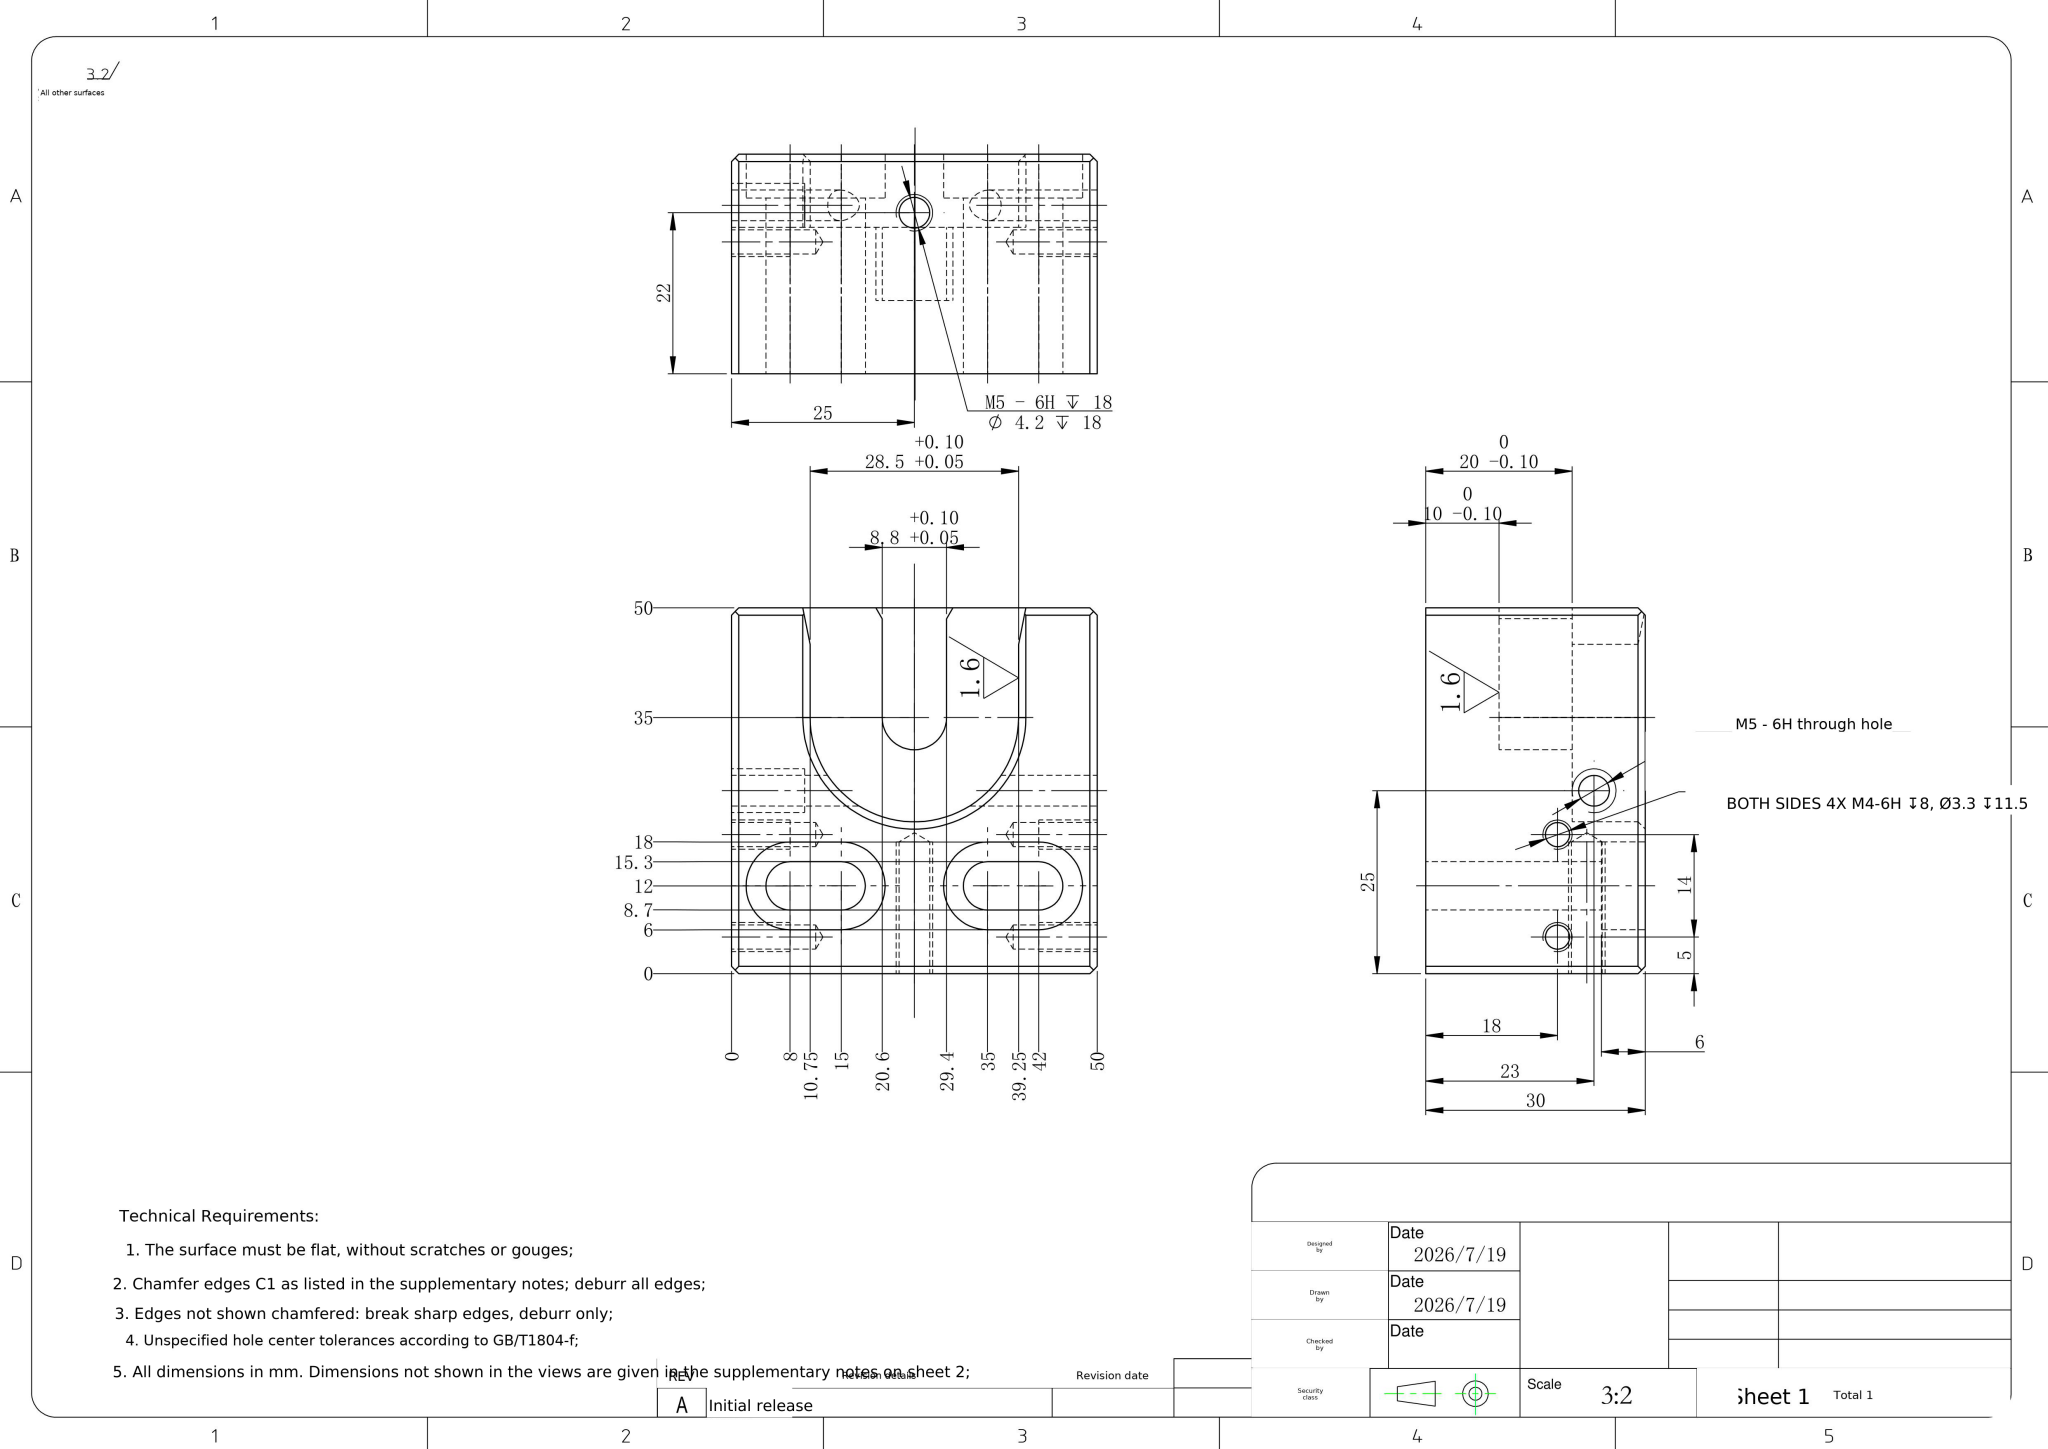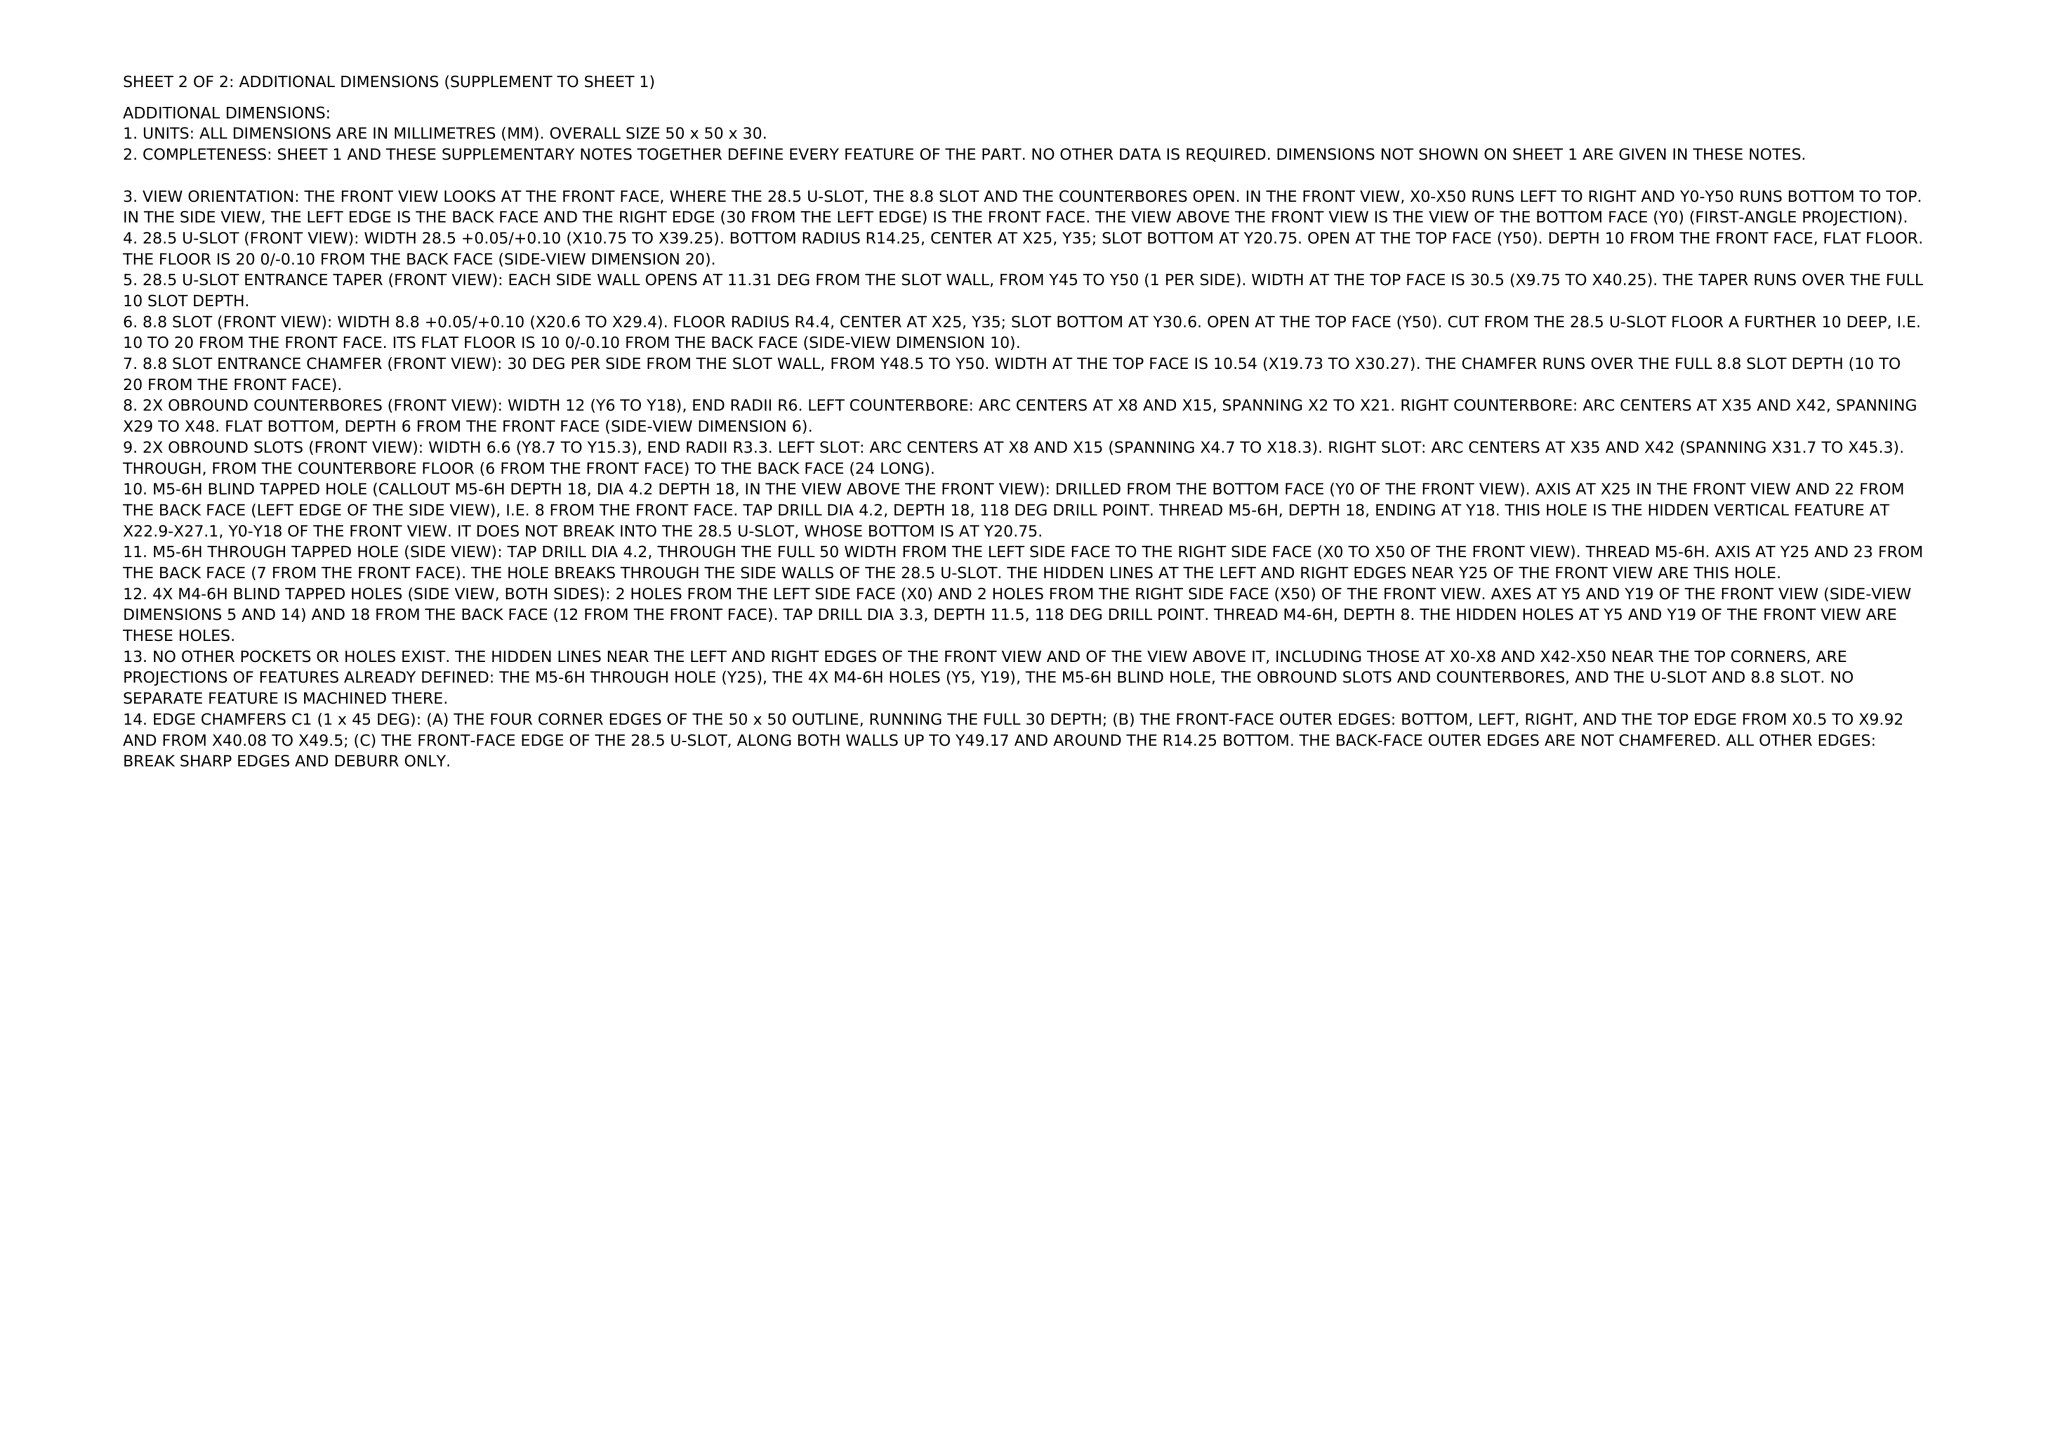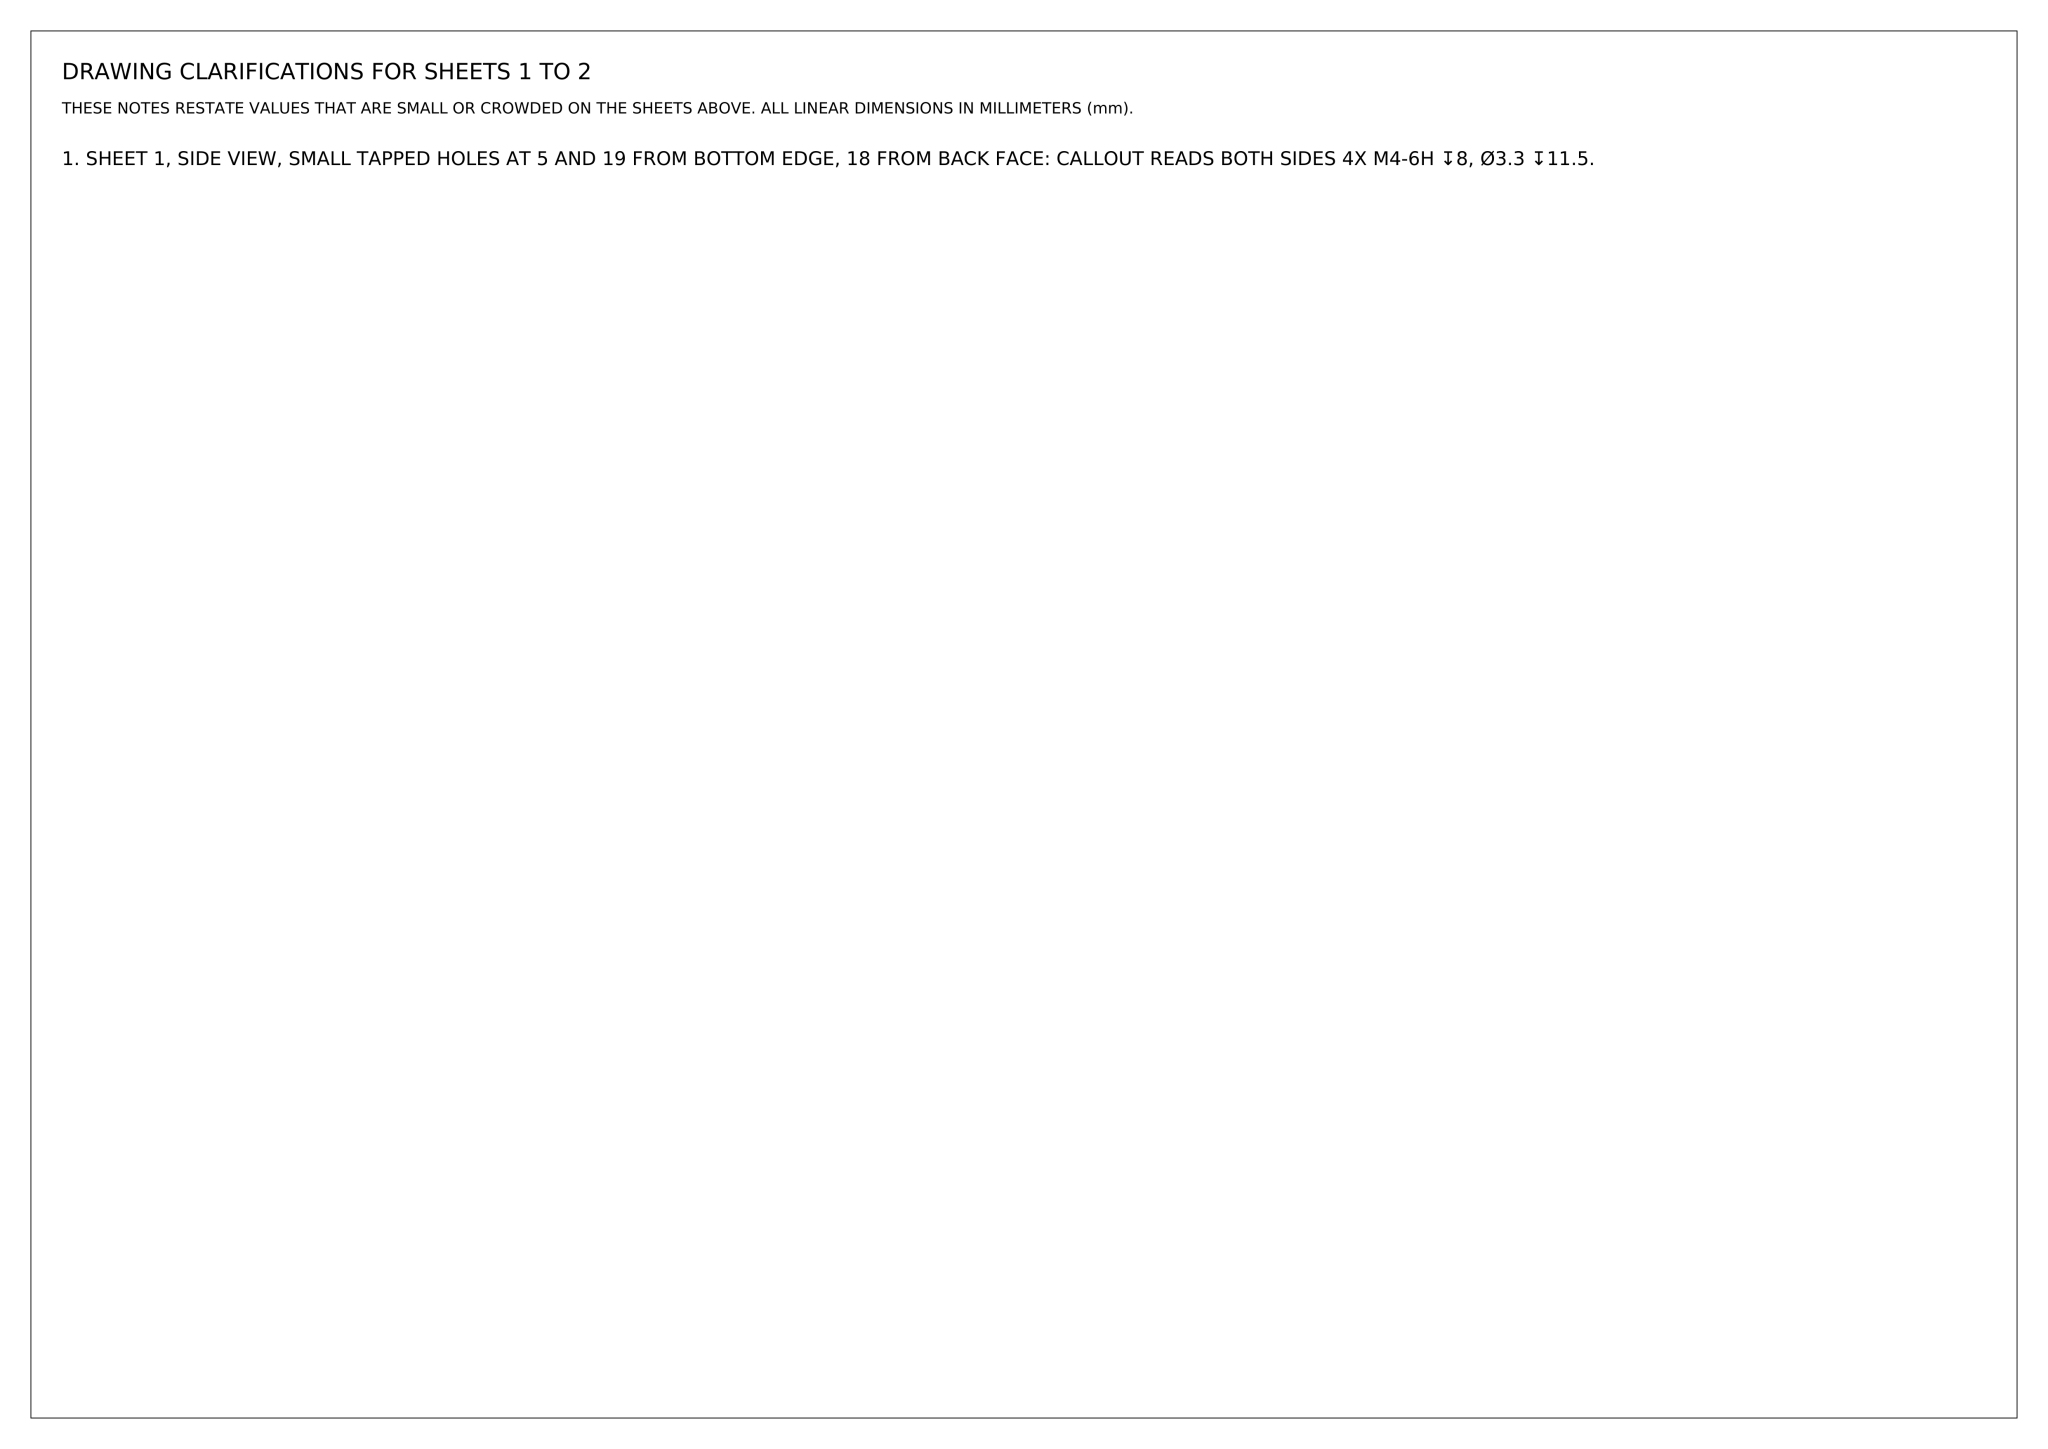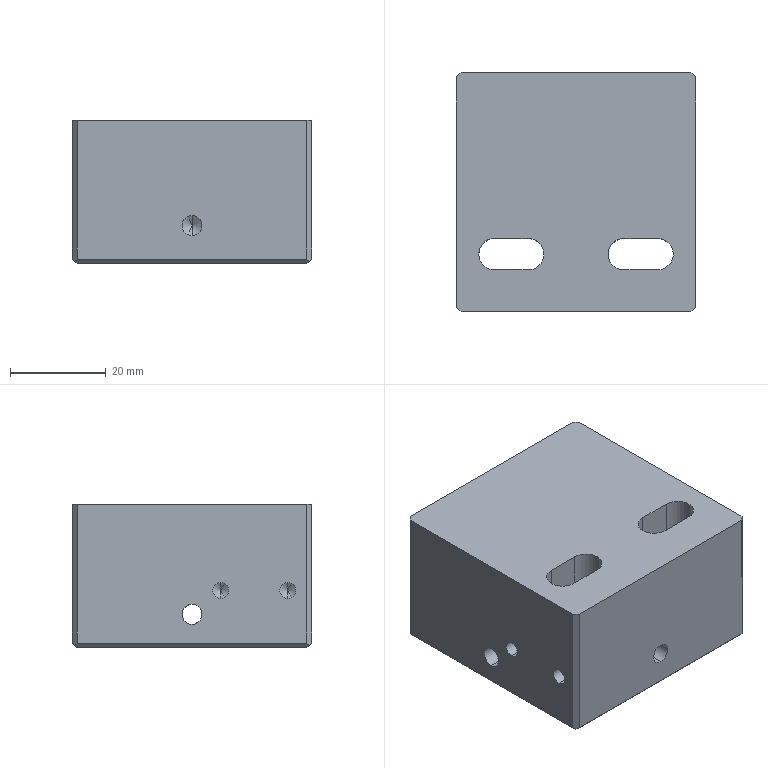Part | NX | mm | 1 solid | 76 faces | box 50 x 50 x 30 mm | volume 58372 mm3 | plane 37 | cylinder 28 | cone 11 | commonest cylinder face diameters 3.3 x8 6.6 x6 12 x6 4.2 x6 28.5 x1 8.8 x1